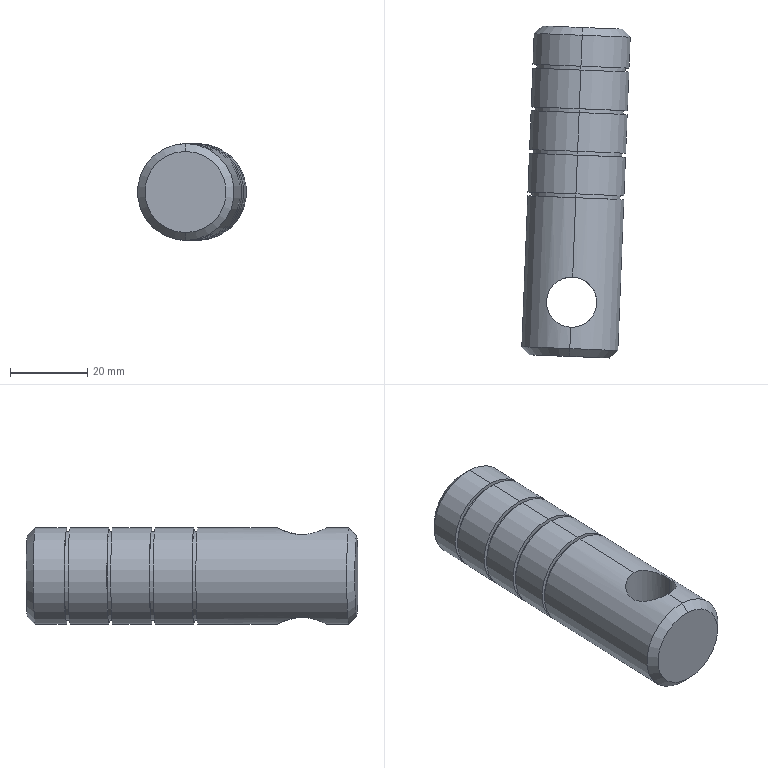Component | SolidWorks | Plunger-1 | 1 solid | 36 faces | volume 37923 mm3 | cylinder 22 | plane 10 | cone 4 | commonest cylinder face diameters 25 x10 23 x8 13 x4